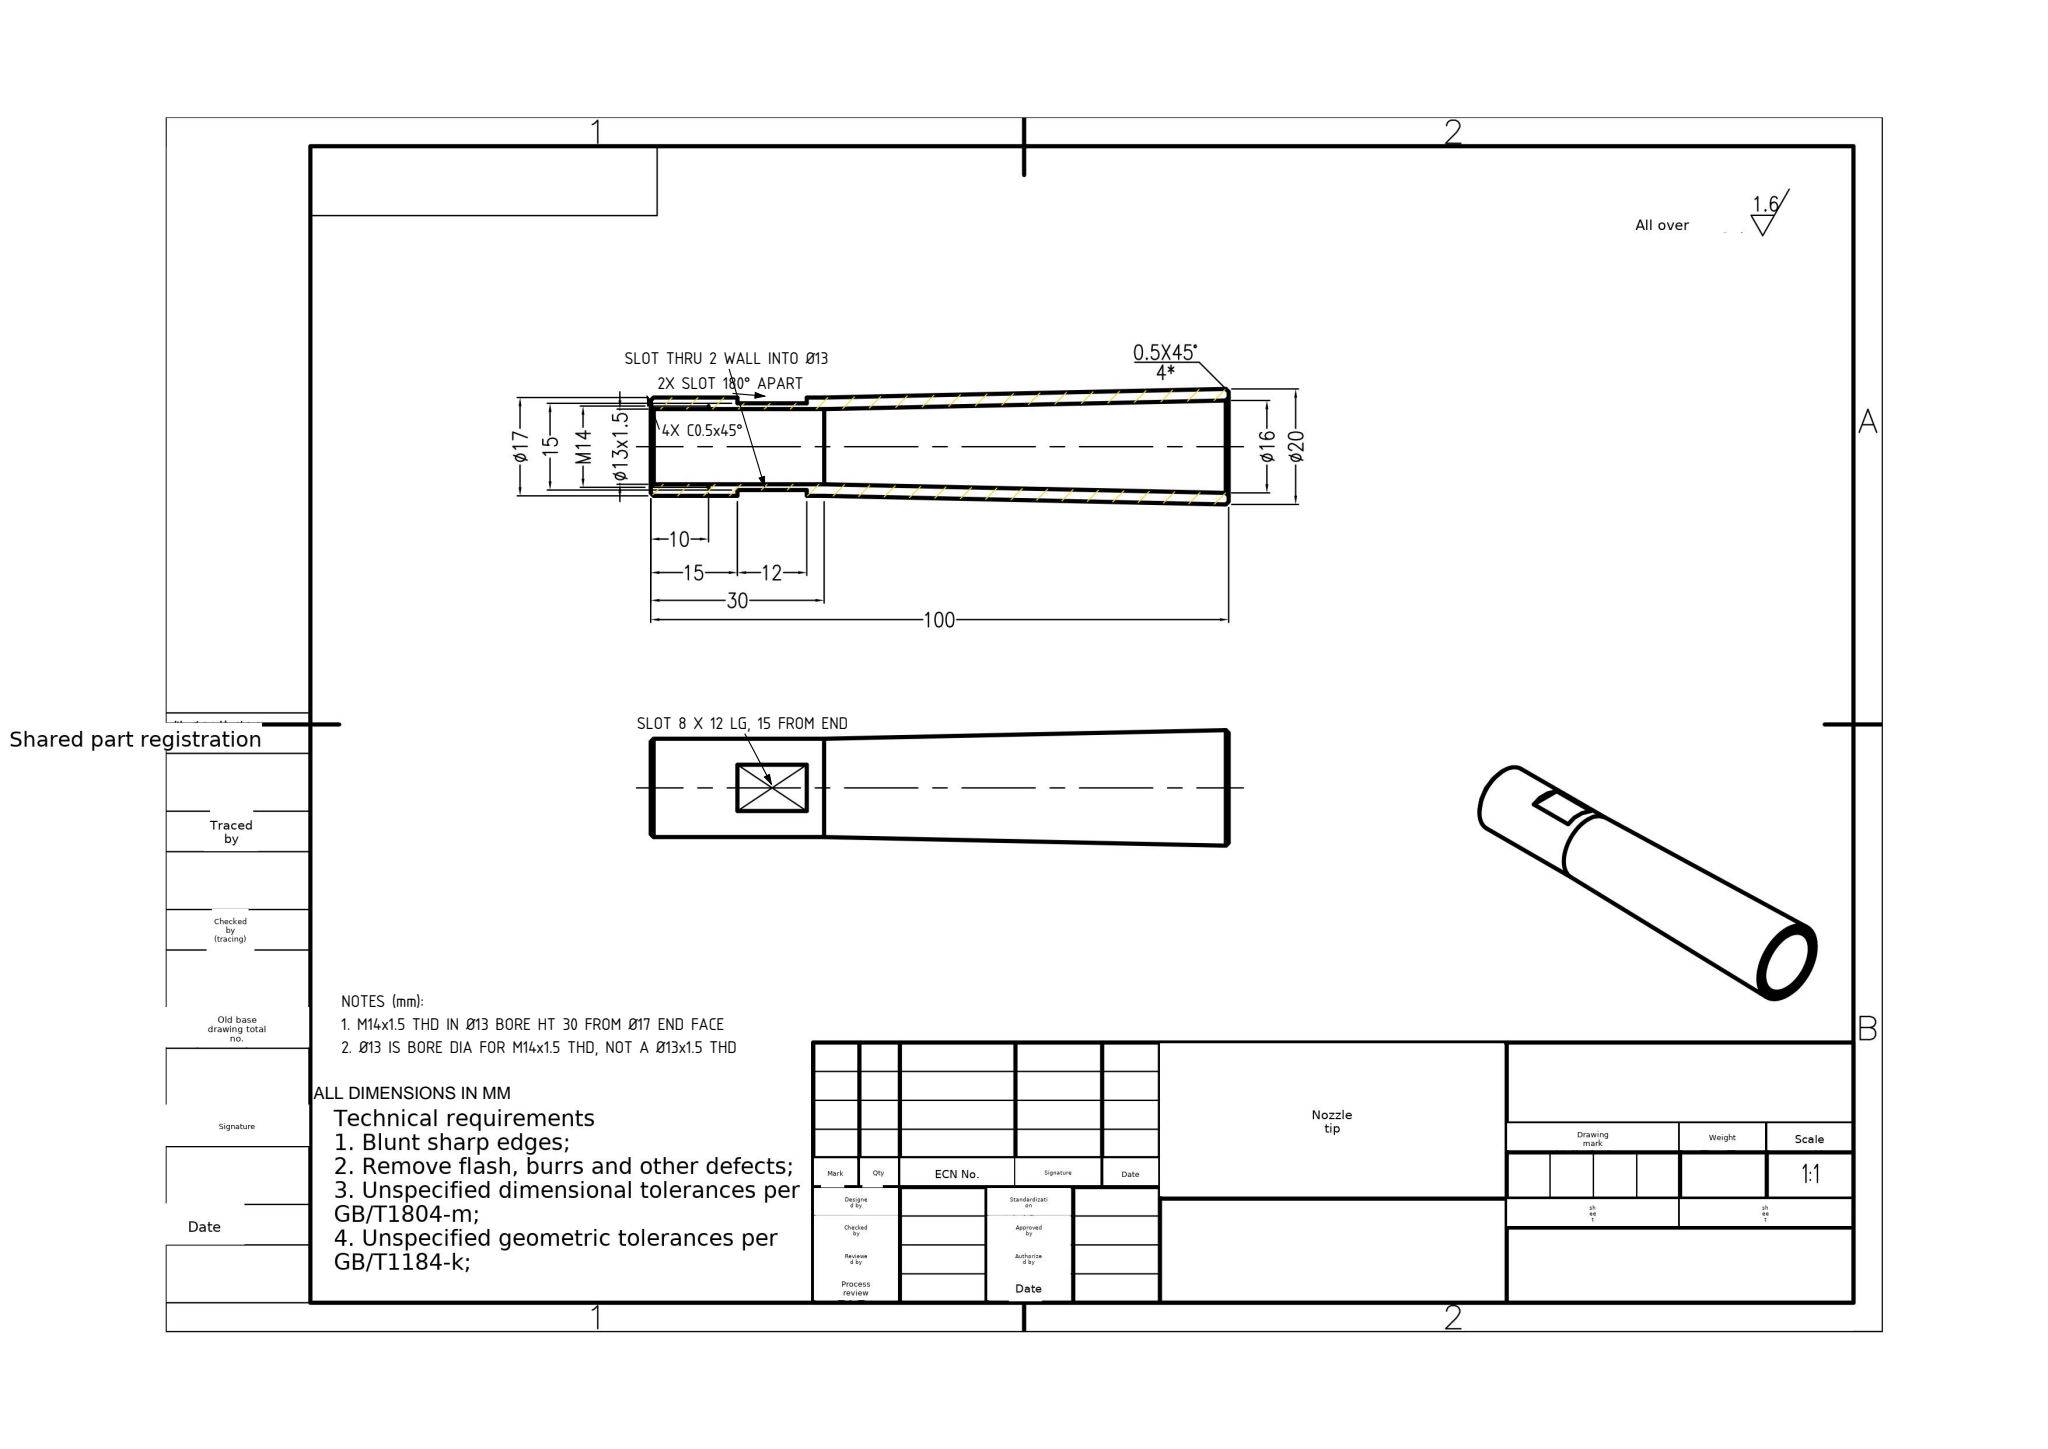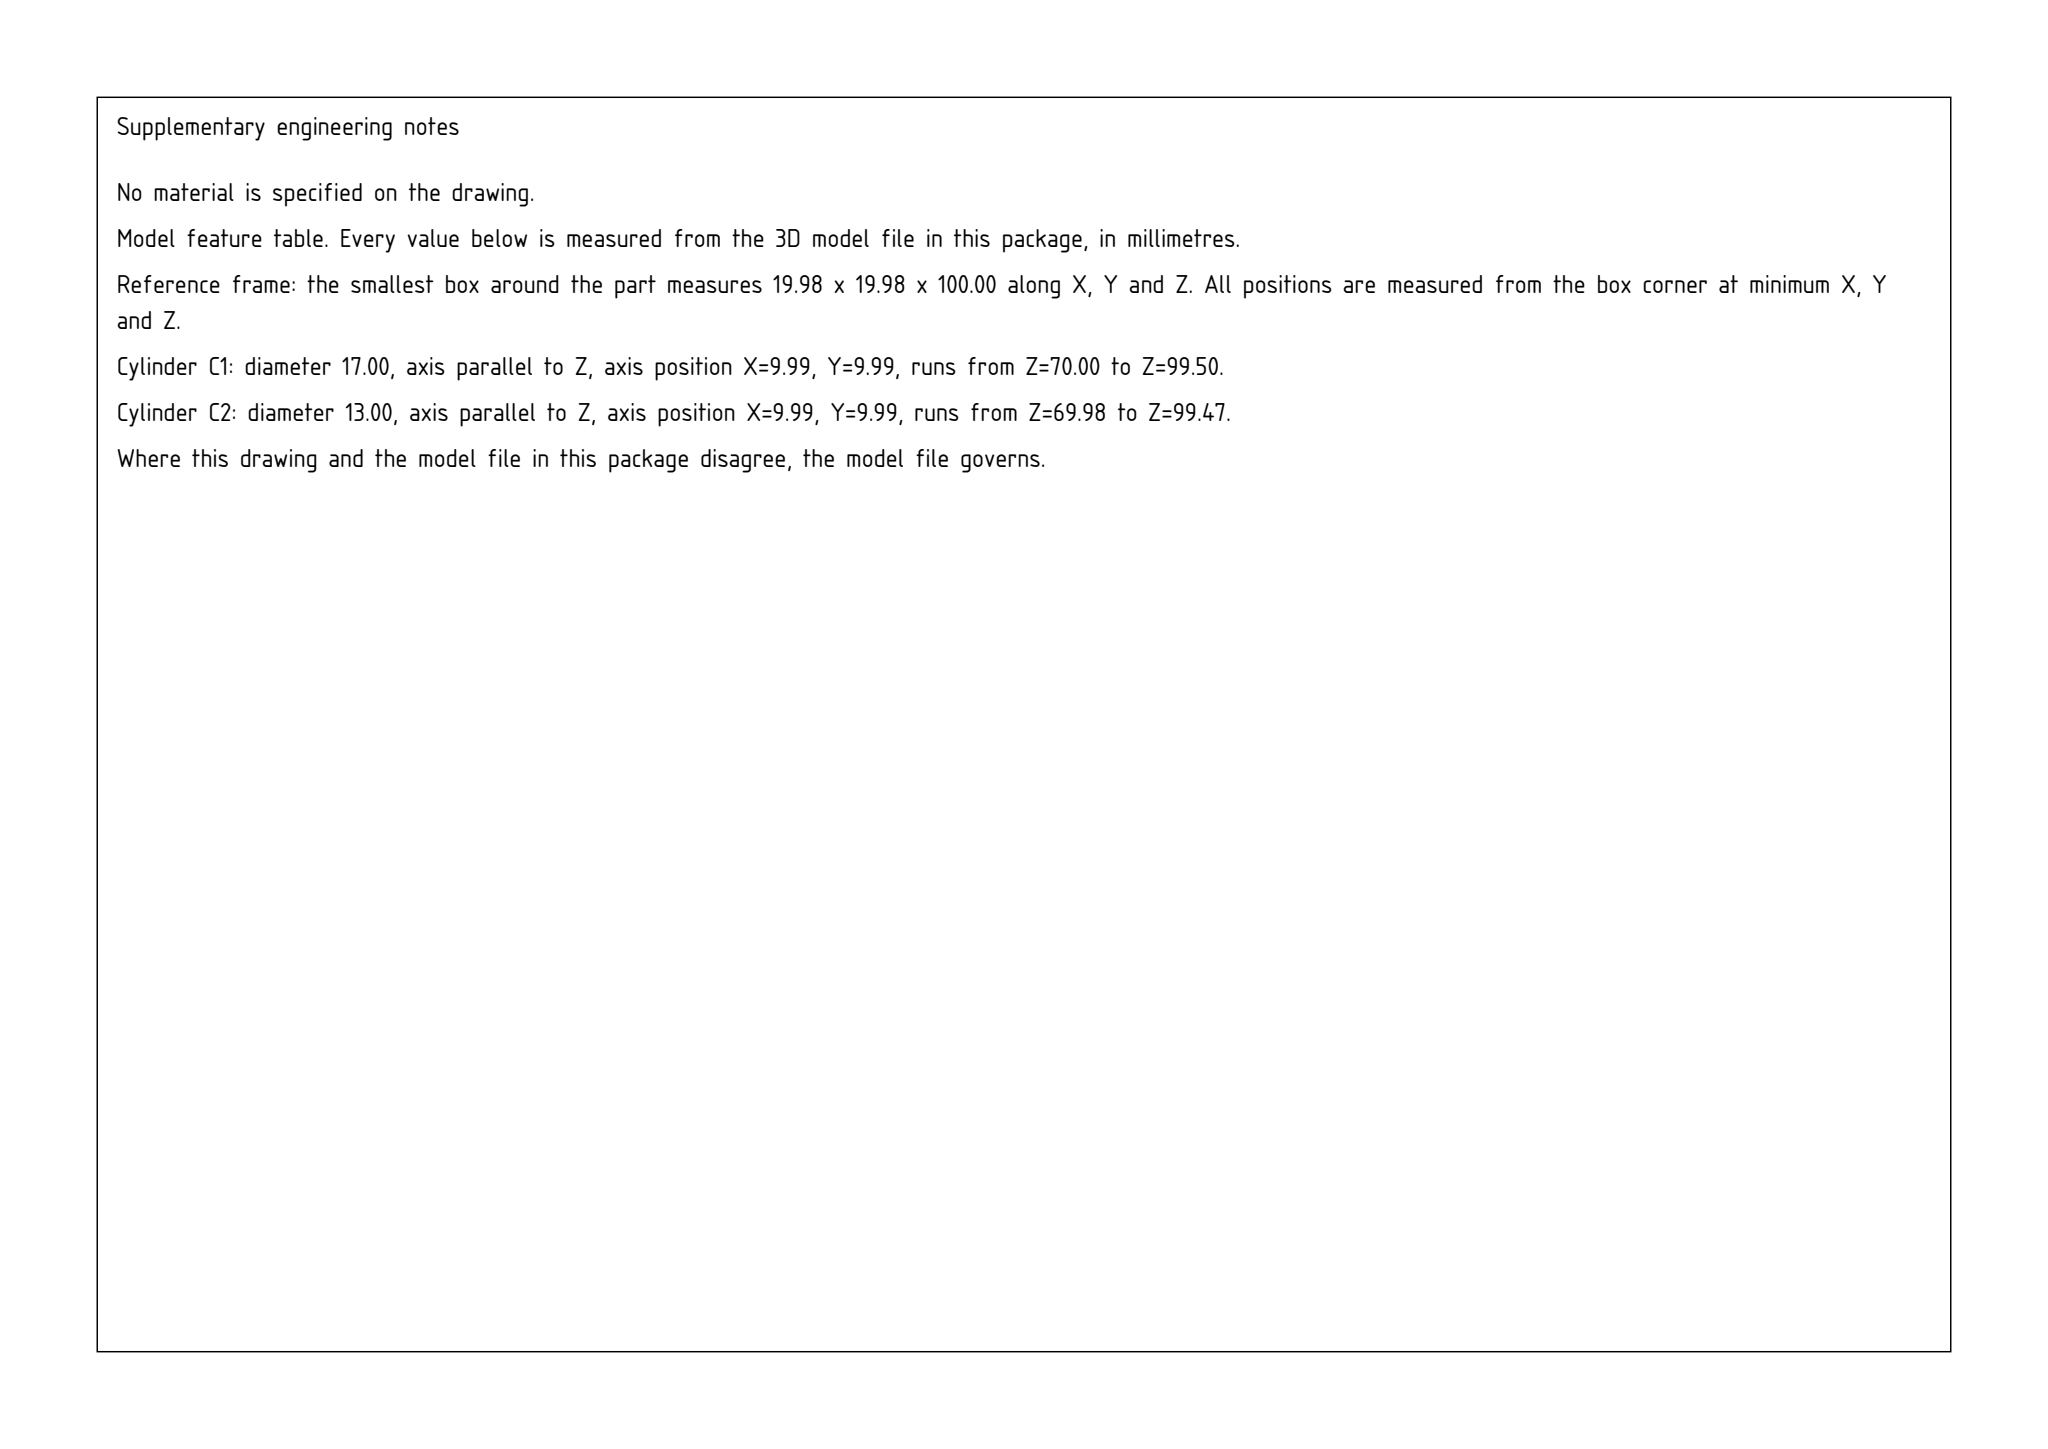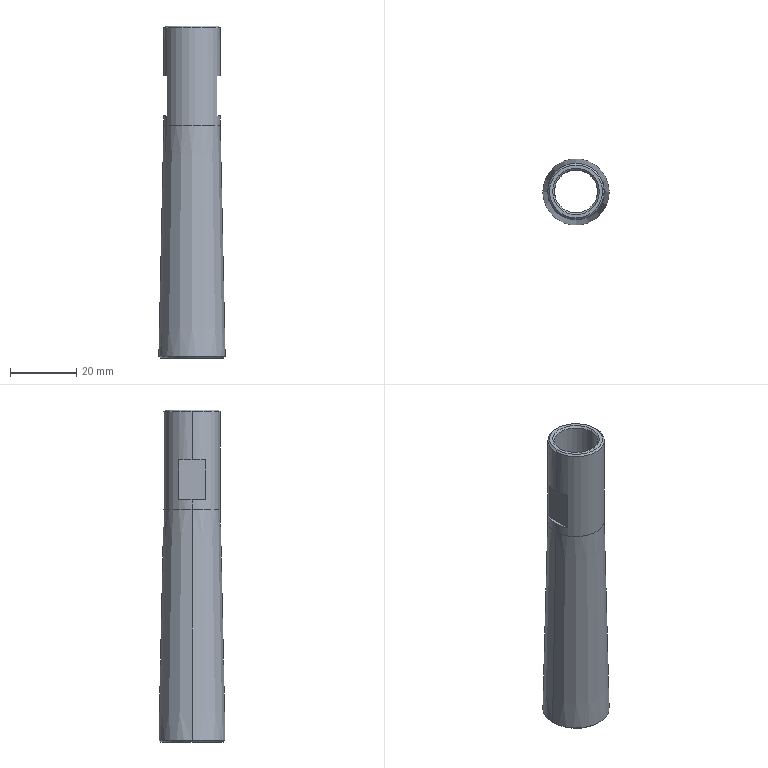Part | SolidWorks | mm | 1 solid | 24 faces | box 19.98 x 19.98 x 100 mm | volume 9930 mm3 | cone 12 | plane 8 | cylinder 4 | commonest cylinder face diameters 13 x2 17 x2
Drawing notes:
RECT SLOT 8 WIDE x 12 LG ON Ø17, 15 FROM Ø17 END FACE | from the solid: Planes x=2.5 & x=17.5, y 6-14 (8 wide), z 73-85 (12 lg); z=100 end face minus 85 = 15
SLOT: 2 PLCS, 180° APART ON Ø17 | from the solid: Two parallel slot walls at x=2.5 and x=17.5, both y 6-14, z 73-85, about axis x=y=10
SLOTS THRU 2 THK WALL INTO Ø13 BORE | from the solid: Ø17 OD and Ø13 bore (z 70-99.5) give 2 wall; slot end faces span x 1.5-2.5 and 17.5-18.5
M14x1.5 THD IN Ø13 BORE HT 30 FROM Ø17 END FACE | from the solid: hole/bore Ø13 z=70 to 99.5 with 0.5 chamfer to end face z=100; depth from face = 30
C0.5 x 45° 4 PLCS: OD & BORE, BOTH ENDS | from the solid: 90° cones ref Ø16 & Ø14.05 at z 99.5-100 and Ø19.98 & Ø17.02 at z 0-0.5, each 0.5 long
Ø13 IS BORE DIA FOR M14x1.5 THD, NOT A Ø13x1.5 THD | from the solid: Single cylindrical bore Ø13.0, z 70-99.5, no second thread feature in model
build123d program:
from build123d import *
from OCP.BRepFilletAPI import BRepFilletAPI_MakeChamfer

# Parameters (mm, degrees)
CUT_EXTRUDE2_DEPTH           = 20
CUT_EXTRUDE2_DEPTH_BACK      = 20
SKETCH4_W                    = 4.877
SKETCH4_H                    = 12
SKETCH4_W_2                  = 5.828
M14_TAPPED_HOLE1_D           = 12
M14_TAPPED_HOLE1_DEPTH       = 10
M14_TAPPED_HOLE1_CSINK_D     = 14.05
M14_TAPPED_HOLE1_CSINK_ANGLE = 90
M14_TAPPED_HOLE1_TIP         = 3.605
CHAMFER1_SIZE                = 0.5
CHAMFER1_SIZE2               = 0.5111
CHAMFER1_SIZE2_2             = 0.4896


with BuildPart() as part:
    # Sketch3 → Revolve1 (revolve)
    with BuildSketch(Plane(origin=(0, 0, 0), x_dir=(0, 0, -1), z_dir=(1, 0, 0)), mode=Mode.PRIVATE) as revolve1_sk:
        Polygon((0, 6.5), (0, 8.5), (30, 8.5), (100, 10), (100, 8), (30.021, 6.5), align=None)
    revolve(revolve1_sk.sketch.rotate(Axis((0, 0, 20.221), (0, 0, -1)), 90), axis=Axis((0, 0, 20.221), (0, 0, -1)))

    # Sketch4 → Cut-Extrude2 (cut, two sides: drawn at the far end of the back side and taken through both)
    with BuildSketch(Plane(origin=(0, 0, 0), x_dir=(1, 0, 0), z_dir=(0, 1, 0)).offset(-CUT_EXTRUDE2_DEPTH_BACK)):
        with Locations((-9.939, 21)):
            Rectangle(SKETCH4_W, SKETCH4_H)
        with Locations((10.414, 21)):
            Rectangle(SKETCH4_W_2, SKETCH4_H)
    extrude(amount=CUT_EXTRUDE2_DEPTH + CUT_EXTRUDE2_DEPTH_BACK, mode=Mode.SUBTRACT)

    # M14 Tapped Hole1
    with Locations(Plane.XY):
        with Locations((0, 0)):
            CounterSinkHole(M14_TAPPED_HOLE1_D / 2, M14_TAPPED_HOLE1_CSINK_D / 2, depth=M14_TAPPED_HOLE1_DEPTH, counter_sink_angle=M14_TAPPED_HOLE1_CSINK_ANGLE)
            with Locations((0, 0, -(M14_TAPPED_HOLE1_DEPTH + M14_TAPPED_HOLE1_TIP / 2))):  # 118° drill point
                Cone(0, M14_TAPPED_HOLE1_D / 2, M14_TAPPED_HOLE1_TIP, mode=Mode.SUBTRACT)

    # Chamfer1: one chamfer whose edges measure the first distance from different faces: ONE call of the kernel's chamfer builder (chamfer() names one face for all edges)
    chamfer1_edges_1 = [part.edges().sort_by_distance(p)[0] for p in [
        (-8.5, 0, 0),
    ]]
    chamfer1_edges_2 = [part.edges().sort_by_distance(p)[0] for p in [
        (-8, 0, -100),
    ]]
    chamfer1_side_2 = [part.faces().sort_by_distance(p)[0] for p in [
        (-7.25, 0, -65.011),
    ]]
    chamfer1_edges_3 = [part.edges().sort_by_distance(p)[0] for p in [
        (-10, 0, -100),
    ]]
    chamfer1_side_3 = [part.faces().sort_by_distance(p)[0] for p in [
        (-9.717, 0, -100),
    ]]
    chamfer1 = BRepFilletAPI_MakeChamfer(part.part.solid().wrapped)
    for e in chamfer1_edges_1:
        chamfer1.Add(CHAMFER1_SIZE, e.wrapped)
    for e in chamfer1_edges_2:
        chamfer1.Add(CHAMFER1_SIZE, CHAMFER1_SIZE2, e.wrapped, chamfer1_side_2[0].wrapped)  # the first distance lies on this face
    for e in chamfer1_edges_3:
        chamfer1.Add(CHAMFER1_SIZE, CHAMFER1_SIZE2_2, e.wrapped, chamfer1_side_3[0].wrapped)  # the first distance lies on this face
    add(Compound.cast(chamfer1.Shape()), mode=Mode.REPLACE)


solid = part.part
STEP:
#1=CARTESIAN_POINT('',(8.,0.,0.));
#2=VERTEX_POINT('',#1);
#3=CARTESIAN_POINT('',(-8.,0.,0.));
#4=VERTEX_POINT('',#3);
#5=CARTESIAN_POINT('',(0.,0.,0.));
#6=DIRECTION('',(0.,0.,1.));
#7=DIRECTION('',(-1.,0.,0.));
#8=AXIS2_PLACEMENT_3D('',#5,#6,#7);
#9=CIRCLE('',#8,8.);
#10=EDGE_CURVE('',#2,#4,#9,.T.);
#11=ORIENTED_EDGE('',*,*,#10,.F.);
#12=CARTESIAN_POINT('',(8.5,0.,-0.5));
#13=VERTEX_POINT('',#12);
#14=CARTESIAN_POINT('',(8.,0.,0.));
#15=DIRECTION('',(0.7071,0.,-0.7071));
#16=VECTOR('',#15,1000.);
#17=LINE('',#14,#16);
#18=EDGE_CURVE('',#2,#13,#17,.T.);
#19=ORIENTED_EDGE('',*,*,#18,.T.);
#20=CARTESIAN_POINT('',(-8.5,0.,-0.5));
#21=VERTEX_POINT('',#20);
#22=CARTESIAN_POINT('',(0.,0.,-0.5));
#23=DIRECTION('',(0.,0.,-1.));
#24=DIRECTION('',(-1.,0.,0.));
#25=AXIS2_PLACEMENT_3D('',#22,#23,#24);
#26=CIRCLE('',#25,8.5);
#27=EDGE_CURVE('',#21,#13,#26,.T.);
#28=ORIENTED_EDGE('',*,*,#27,.F.);
#29=CARTESIAN_POINT('',(-8.,0.,0.));
#30=DIRECTION('',(-0.7071,0.,-0.7071));
#31=VECTOR('',#30,1000.);
#32=LINE('',#29,#31);
#33=EDGE_CURVE('',#4,#21,#32,.T.);
#34=ORIENTED_EDGE('',*,*,#33,.F.);
#35=EDGE_LOOP('',(#11,#19,#28,#34));
#36=FACE_OUTER_BOUND('',#35,.T.);
#37=CARTESIAN_POINT('',(0.,0.,0.));
#38=DIRECTION('',(0.,0.,-1.));
#39=DIRECTION('',(-1.,0.,0.));
#40=AXIS2_PLACEMENT_3D('',#37,#38,#39);
#41=CONICAL_SURFACE('',#40,8.,0.7854);
#42=ADVANCED_FACE('',(#36),#41,.T.);
#43=CARTESIAN_POINT('',(-9.5,0.,-100.));
#44=VERTEX_POINT('',#43);
#45=CARTESIAN_POINT('',(9.5,0.,-100.));
#46=VERTEX_POINT('',#45);
#47=CARTESIAN_POINT('',(0.,0.,-100.));
#48=DIRECTION('',(0.,0.,-1.));
#49=DIRECTION('',(1.,0.,0.));
#50=AXIS2_PLACEMENT_3D('',#47,#48,#49);
#51=CIRCLE('',#50,9.5);
#52=EDGE_CURVE('',#44,#46,#51,.T.);
#53=ORIENTED_EDGE('',*,*,#52,.F.);
#54=CARTESIAN_POINT('',(-9.99,0.,-99.51));
#55=VERTEX_POINT('',#54);
#56=CARTESIAN_POINT('',(-9.99,0.,-99.51));
#57=DIRECTION('',(-0.7071,0.,0.7071));
#58=VECTOR('',#57,1000.);
#59=LINE('',#56,#58);
#60=EDGE_CURVE('',#44,#55,#59,.T.);
#61=ORIENTED_EDGE('',*,*,#60,.T.);
#62=CARTESIAN_POINT('',(9.99,0.,-99.51));
#63=VERTEX_POINT('',#62);
#64=CARTESIAN_POINT('',(0.,0.,-99.51));
#65=DIRECTION('',(0.,0.,1.));
#66=DIRECTION('',(1.,0.,0.));
#67=AXIS2_PLACEMENT_3D('',#64,#65,#66);
#68=CIRCLE('',#67,9.99);
#69=EDGE_CURVE('',#63,#55,#68,.T.);
#70=ORIENTED_EDGE('',*,*,#69,.F.);
#71=CARTESIAN_POINT('',(9.99,0.,-99.51));
#72=DIRECTION('',(0.7071,0.,0.7071));
#73=VECTOR('',#72,1000.);
#74=LINE('',#71,#73);
#75=EDGE_CURVE('',#46,#63,#74,.T.);
#76=ORIENTED_EDGE('',*,*,#75,.F.);
#77=EDGE_LOOP('',(#53,#61,#70,#76));
#78=FACE_OUTER_BOUND('',#77,.T.);
#79=CARTESIAN_POINT('',(0.,0.,-99.51));
#80=DIRECTION('',(0.,0.,1.));
#81=DIRECTION('',(1.,0.,0.));
#82=AXIS2_PLACEMENT_3D('',#79,#80,#81);
#83=CONICAL_SURFACE('',#82,9.99,0.7854);
#84=ADVANCED_FACE('',(#78),#83,.T.);
#85=CARTESIAN_POINT('',(7.989,0.,-99.5));
#86=VERTEX_POINT('',#85);
#87=CARTESIAN_POINT('',(-7.989,0.,-99.5));
#88=VERTEX_POINT('',#87);
#89=CARTESIAN_POINT('',(0.,0.,-99.5));
#90=DIRECTION('',(0.,0.,-1.));
#91=DIRECTION('',(1.,0.,0.));
#92=AXIS2_PLACEMENT_3D('',#89,#90,#91);
#93=CIRCLE('',#92,7.989);
#94=EDGE_CURVE('',#86,#88,#93,.T.);
#95=ORIENTED_EDGE('',*,*,#94,.F.);
#96=CARTESIAN_POINT('',(8.511,0.,-100.));
#97=VERTEX_POINT('',#96);
#98=CARTESIAN_POINT('',(8.511,0.,-100.));
#99=DIRECTION('',(0.7221,0.,-0.6918));
#100=VECTOR('',#99,1000.);
#101=LINE('',#98,#100);
#102=EDGE_CURVE('',#86,#97,#101,.T.);
#103=ORIENTED_EDGE('',*,*,#102,.T.);
#104=CARTESIAN_POINT('',(-8.511,0.,-100.));
#105=VERTEX_POINT('',#104);
#106=CARTESIAN_POINT('',(0.,0.,-100.));
#107=DIRECTION('',(0.,0.,1.));
#108=DIRECTION('',(1.,0.,0.));
#109=AXIS2_PLACEMENT_3D('',#106,#107,#108);
#110=CIRCLE('',#109,8.511);
#111=EDGE_CURVE('',#105,#97,#110,.T.);
#112=ORIENTED_EDGE('',*,*,#111,.F.);
#113=CARTESIAN_POINT('',(-8.511,0.,-100.));
#114=DIRECTION('',(-0.7221,0.,-0.6918));
#115=VECTOR('',#114,1000.);
#116=LINE('',#113,#115);
#117=EDGE_CURVE('',#88,#105,#116,.T.);
#118=ORIENTED_EDGE('',*,*,#117,.F.);
#119=EDGE_LOOP('',(#95,#103,#112,#118));
#120=FACE_OUTER_BOUND('',#119,.T.);
#121=CARTESIAN_POINT('',(0.,0.,-100.));
#122=DIRECTION('',(0.,0.,-1.));
#123=DIRECTION('',(-1.,0.,0.));
#124=AXIS2_PLACEMENT_3D('',#121,#122,#123);
#125=CONICAL_SURFACE('',#124,8.511,0.8068);
#126=ADVANCED_FACE('',(#120),#125,.F.);
#127=CARTESIAN_POINT('',(-6.5,0.,-0.525));
#128=VERTEX_POINT('',#127);
#129=CARTESIAN_POINT('',(6.5,0.,-0.525));
#130=VERTEX_POINT('',#129);
#131=CARTESIAN_POINT('',(0.,0.,-0.525));
#132=DIRECTION('',(0.,0.,1.));
#133=DIRECTION('',(1.,0.,0.));
#134=AXIS2_PLACEMENT_3D('',#131,#132,#133);
#135=CIRCLE('',#134,6.5);
#136=EDGE_CURVE('',#128,#130,#135,.T.);
#137=ORIENTED_EDGE('',*,*,#136,.F.);
#138=CARTESIAN_POINT('',(-7.025,0.,-0.));
#139=VERTEX_POINT('',#138);
#140=CARTESIAN_POINT('',(-7.025,0.,-0.));
#141=DIRECTION('',(-0.7071,0.,0.7071));
#142=VECTOR('',#141,1000.);
#143=LINE('',#140,#142);
#144=EDGE_CURVE('',#128,#139,#143,.T.);
#145=ORIENTED_EDGE('',*,*,#144,.T.);
#146=CARTESIAN_POINT('',(7.025,0.,-0.));
#147=VERTEX_POINT('',#146);
#148=CARTESIAN_POINT('',(0.,0.,-0.));
#149=DIRECTION('',(0.,0.,1.));
#150=DIRECTION('',(1.,0.,0.));
#151=AXIS2_PLACEMENT_3D('',#148,#149,#150);
#152=CIRCLE('',#151,7.025);
#153=EDGE_CURVE('',#139,#147,#152,.T.);
#154=ORIENTED_EDGE('',*,*,#153,.T.);
#155=CARTESIAN_POINT('',(7.025,0.,-0.));
#156=DIRECTION('',(0.7071,0.,0.7071));
#157=VECTOR('',#156,1000.);
#158=LINE('',#155,#157);
#159=EDGE_CURVE('',#130,#147,#158,.T.);
#160=ORIENTED_EDGE('',*,*,#159,.F.);
#161=EDGE_LOOP('',(#137,#145,#154,#160));
#162=FACE_OUTER_BOUND('',#161,.T.);
#163=CARTESIAN_POINT('',(0.,0.,-0.));
#164=DIRECTION('',(0.,0.,1.));
#165=DIRECTION('',(1.,0.,0.));
#166=AXIS2_PLACEMENT_3D('',#163,#164,#165);
#167=CONICAL_SURFACE('',#166,7.025,0.7854);
#168=ADVANCED_FACE('',(#162),#167,.F.);
#169=CARTESIAN_POINT('',(-6.5,0.,-30.021));
#170=VERTEX_POINT('',#169);
#171=CARTESIAN_POINT('',(6.5,0.,-30.021));
#172=VERTEX_POINT('',#171);
#173=CARTESIAN_POINT('',(0.,0.,-30.021));
#174=DIRECTION('',(0.,0.,1.));
#175=DIRECTION('',(1.,0.,0.));
#176=AXIS2_PLACEMENT_3D('',#173,#174,#175);
#177=CIRCLE('',#176,6.5);
#178=EDGE_CURVE('',#170,#172,#177,.T.);
#179=ORIENTED_EDGE('',*,*,#178,.F.);
#180=CARTESIAN_POINT('',(-6.5,0.,20.221));
#181=DIRECTION('',(0.,0.,1.));
#182=VECTOR('',#181,1000.);
#183=LINE('',#180,#182);
#184=EDGE_CURVE('',#170,#128,#183,.T.);
#185=ORIENTED_EDGE('',*,*,#184,.T.);
#186=ORIENTED_EDGE('',*,*,#136,.T.);
#187=CARTESIAN_POINT('',(6.5,0.,20.221));
#188=DIRECTION('',(0.,0.,1.));
#189=VECTOR('',#188,1000.);
#190=LINE('',#187,#189);
#191=EDGE_CURVE('',#172,#130,#190,.T.);
#192=ORIENTED_EDGE('',*,*,#191,.F.);
#193=EDGE_LOOP('',(#179,#185,#186,#192));
#194=FACE_OUTER_BOUND('',#193,.T.);
#195=CARTESIAN_POINT('',(0.,0.,20.221));
#196=DIRECTION('',(0.,0.,1.));
#197=DIRECTION('',(1.,0.,0.));
#198=AXIS2_PLACEMENT_3D('',#195,#196,#197);
#199=CYLINDRICAL_SURFACE('',#198,6.5);
#200=ADVANCED_FACE('',(#194),#199,.F.);
#201=ORIENTED_EDGE('',*,*,#178,.T.);
#202=CARTESIAN_POINT('',(6.5,0.,-30.021));
#203=DIRECTION('',(0.02142,0.,-0.9998));
#204=VECTOR('',#203,1000.);
#205=LINE('',#202,#204);
#206=EDGE_CURVE('',#172,#86,#205,.T.);
#207=ORIENTED_EDGE('',*,*,#206,.T.);
#208=ORIENTED_EDGE('',*,*,#94,.T.);
#209=CARTESIAN_POINT('',(-6.5,0.,-30.021));
#210=DIRECTION('',(-0.02142,0.,-0.9998));
#211=VECTOR('',#210,1000.);
#212=LINE('',#209,#211);
#213=EDGE_CURVE('',#170,#88,#212,.T.);
#214=ORIENTED_EDGE('',*,*,#213,.F.);
#215=EDGE_LOOP('',(#201,#207,#208,#214));
#216=FACE_OUTER_BOUND('',#215,.T.);
#217=CARTESIAN_POINT('',(0.,0.,-30.021));
#218=DIRECTION('',(0.,0.,-1.));
#219=DIRECTION('',(-1.,0.,0.));
#220=AXIS2_PLACEMENT_3D('',#217,#218,#219);
#221=CONICAL_SURFACE('',#220,6.5,0.02143);
#222=ADVANCED_FACE('',(#216),#221,.F.);
#223=CARTESIAN_POINT('',(8.5,0.,-30.));
#224=VERTEX_POINT('',#223);
#225=CARTESIAN_POINT('',(-8.5,0.,-30.));
#226=VERTEX_POINT('',#225);
#227=CARTESIAN_POINT('',(0.,0.,-30.));
#228=DIRECTION('',(0.,0.,1.));
#229=DIRECTION('',(1.,0.,0.));
#230=AXIS2_PLACEMENT_3D('',#227,#228,#229);
#231=CIRCLE('',#230,8.5);
#232=EDGE_CURVE('',#224,#226,#231,.T.);
#233=ORIENTED_EDGE('',*,*,#232,.F.);
#234=CARTESIAN_POINT('',(10.,0.,-100.));
#235=DIRECTION('',(0.02142,0.,-0.9998));
#236=VECTOR('',#235,1000.);
#237=LINE('',#234,#236);
#238=EDGE_CURVE('',#224,#63,#237,.T.);
#239=ORIENTED_EDGE('',*,*,#238,.T.);
#240=ORIENTED_EDGE('',*,*,#69,.T.);
#241=CARTESIAN_POINT('',(-10.,0.,-100.));
#242=DIRECTION('',(-0.02142,0.,-0.9998));
#243=VECTOR('',#242,1000.);
#244=LINE('',#241,#243);
#245=EDGE_CURVE('',#226,#55,#244,.T.);
#246=ORIENTED_EDGE('',*,*,#245,.F.);
#247=EDGE_LOOP('',(#233,#239,#240,#246));
#248=FACE_OUTER_BOUND('',#247,.T.);
#249=CARTESIAN_POINT('',(0.,0.,-100.));
#250=DIRECTION('',(0.,0.,-1.));
#251=DIRECTION('',(-1.,0.,0.));
#252=AXIS2_PLACEMENT_3D('',#249,#250,#251);
#253=CONICAL_SURFACE('',#252,10.,0.02143);
#254=ADVANCED_FACE('',(#248),#253,.T.);
#255=ORIENTED_EDGE('',*,*,#232,.T.);
#256=CARTESIAN_POINT('',(-8.5,0.,-27.));
#257=VERTEX_POINT('',#256);
#258=CARTESIAN_POINT('',(-8.5,0.,20.221));
#259=DIRECTION('',(0.,0.,1.));
#260=VECTOR('',#259,1000.);
#261=LINE('',#258,#260);
#262=EDGE_CURVE('',#226,#257,#261,.T.);
#263=ORIENTED_EDGE('',*,*,#262,.T.);
#264=CARTESIAN_POINT('',(-7.5,4.,-27.));
#265=VERTEX_POINT('',#264);
#266=CARTESIAN_POINT('',(0.,0.,-27.));
#267=DIRECTION('',(0.,0.,1.));
#268=DIRECTION('',(1.,0.,-0.));
#269=AXIS2_PLACEMENT_3D('',#266,#267,#268);
#270=CIRCLE('',#269,8.5);
#271=EDGE_CURVE('',#265,#257,#270,.T.);
#272=ORIENTED_EDGE('',*,*,#271,.F.);
#273=CARTESIAN_POINT('',(-7.5,4.,-15.));
#274=VERTEX_POINT('',#273);
#275=CARTESIAN_POINT('',(-7.5,4.,20.221));
#276=DIRECTION('',(0.,0.,-1.));
#277=VECTOR('',#276,1000.);
#278=LINE('',#275,#277);
#279=EDGE_CURVE('',#274,#265,#278,.T.);
#280=ORIENTED_EDGE('',*,*,#279,.F.);
#281=CARTESIAN_POINT('',(-8.5,0.,-15.));
#282=VERTEX_POINT('',#281);
#283=CARTESIAN_POINT('',(0.,0.,-15.));
#284=DIRECTION('',(0.,0.,-1.));
#285=DIRECTION('',(-1.,0.,0.));
#286=AXIS2_PLACEMENT_3D('',#283,#284,#285);
#287=CIRCLE('',#286,8.5);
#288=EDGE_CURVE('',#282,#274,#287,.T.);
#289=ORIENTED_EDGE('',*,*,#288,.F.);
#290=CARTESIAN_POINT('',(-8.5,0.,20.221));
#291=DIRECTION('',(0.,0.,1.));
#292=VECTOR('',#291,1000.);
#293=LINE('',#290,#292);
#294=EDGE_CURVE('',#282,#21,#293,.T.);
#295=ORIENTED_EDGE('',*,*,#294,.T.);
#296=ORIENTED_EDGE('',*,*,#27,.T.);
#297=CARTESIAN_POINT('',(8.5,0.,-15.));
#298=VERTEX_POINT('',#297);
#299=CARTESIAN_POINT('',(8.5,0.,20.221));
#300=DIRECTION('',(0.,0.,1.));
#301=VECTOR('',#300,1000.);
#302=LINE('',#299,#301);
#303=EDGE_CURVE('',#298,#13,#302,.T.);
#304=ORIENTED_EDGE('',*,*,#303,.F.);
#305=CARTESIAN_POINT('',(7.5,4.,-15.));
#306=VERTEX_POINT('',#305);
#307=CARTESIAN_POINT('',(0.,0.,-15.));
#308=DIRECTION('',(0.,0.,-1.));
#309=DIRECTION('',(-1.,0.,0.));
#310=AXIS2_PLACEMENT_3D('',#307,#308,#309);
#311=CIRCLE('',#310,8.5);
#312=EDGE_CURVE('',#306,#298,#311,.T.);
#313=ORIENTED_EDGE('',*,*,#312,.F.);
#314=CARTESIAN_POINT('',(7.5,4.,-27.));
#315=VERTEX_POINT('',#314);
#316=CARTESIAN_POINT('',(7.5,4.,20.221));
#317=DIRECTION('',(0.,0.,1.));
#318=VECTOR('',#317,1000.);
#319=LINE('',#316,#318);
#320=EDGE_CURVE('',#315,#306,#319,.T.);
#321=ORIENTED_EDGE('',*,*,#320,.F.);
#322=CARTESIAN_POINT('',(8.5,0.,-27.));
#323=VERTEX_POINT('',#322);
#324=CARTESIAN_POINT('',(0.,0.,-27.));
#325=DIRECTION('',(0.,0.,1.));
#326=DIRECTION('',(1.,0.,0.));
#327=AXIS2_PLACEMENT_3D('',#324,#325,#326);
#328=CIRCLE('',#327,8.5);
#329=EDGE_CURVE('',#323,#315,#328,.T.);
#330=ORIENTED_EDGE('',*,*,#329,.F.);
#331=CARTESIAN_POINT('',(8.5,0.,20.221));
#332=DIRECTION('',(0.,0.,1.));
#333=VECTOR('',#332,1000.);
#334=LINE('',#331,#333);
#335=EDGE_CURVE('',#224,#323,#334,.T.);
#336=ORIENTED_EDGE('',*,*,#335,.F.);
#337=EDGE_LOOP('',(#255,#263,#272,#280,#289,#295,#296,#304,#313,#321,#330,#336));
#338=FACE_OUTER_BOUND('',#337,.T.);
#339=CARTESIAN_POINT('',(0.,0.,20.221));
#340=DIRECTION('',(0.,0.,1.));
#341=DIRECTION('',(1.,0.,0.));
#342=AXIS2_PLACEMENT_3D('',#339,#340,#341);
#343=CYLINDRICAL_SURFACE('',#342,8.5);
#344=ADVANCED_FACE('',(#338),#343,.T.);
#345=ORIENTED_EDGE('',*,*,#262,.F.);
#346=CARTESIAN_POINT('',(0.,0.,-30.));
#347=DIRECTION('',(0.,0.,1.));
#348=DIRECTION('',(1.,0.,0.));
#349=AXIS2_PLACEMENT_3D('',#346,#347,#348);
#350=CIRCLE('',#349,8.5);
#351=EDGE_CURVE('',#226,#224,#350,.T.);
#352=ORIENTED_EDGE('',*,*,#351,.T.);
#353=ORIENTED_EDGE('',*,*,#335,.T.);
#354=CARTESIAN_POINT('',(7.5,-4.,-27.));
#355=VERTEX_POINT('',#354);
#356=CARTESIAN_POINT('',(0.,0.,-27.));
#357=DIRECTION('',(0.,0.,1.));
#358=DIRECTION('',(1.,0.,0.));
#359=AXIS2_PLACEMENT_3D('',#356,#357,#358);
#360=CIRCLE('',#359,8.5);
#361=EDGE_CURVE('',#355,#323,#360,.T.);
#362=ORIENTED_EDGE('',*,*,#361,.F.);
#363=CARTESIAN_POINT('',(7.5,-4.,-15.));
#364=VERTEX_POINT('',#363);
#365=CARTESIAN_POINT('',(7.5,-4.,20.221));
#366=DIRECTION('',(0.,0.,-1.));
#367=VECTOR('',#366,1000.);
#368=LINE('',#365,#367);
#369=EDGE_CURVE('',#364,#355,#368,.T.);
#370=ORIENTED_EDGE('',*,*,#369,.F.);
#371=CARTESIAN_POINT('',(0.,0.,-15.));
#372=DIRECTION('',(0.,0.,-1.));
#373=DIRECTION('',(-1.,0.,0.));
#374=AXIS2_PLACEMENT_3D('',#371,#372,#373);
#375=CIRCLE('',#374,8.5);
#376=EDGE_CURVE('',#298,#364,#375,.T.);
#377=ORIENTED_EDGE('',*,*,#376,.F.);
#378=ORIENTED_EDGE('',*,*,#303,.T.);
#379=CARTESIAN_POINT('',(0.,0.,-0.5));
#380=DIRECTION('',(0.,0.,-1.));
#381=DIRECTION('',(-1.,0.,0.));
#382=AXIS2_PLACEMENT_3D('',#379,#380,#381);
#383=CIRCLE('',#382,8.5);
#384=EDGE_CURVE('',#13,#21,#383,.T.);
#385=ORIENTED_EDGE('',*,*,#384,.T.);
#386=ORIENTED_EDGE('',*,*,#294,.F.);
#387=CARTESIAN_POINT('',(-7.5,-4.,-15.));
#388=VERTEX_POINT('',#387);
#389=CARTESIAN_POINT('',(0.,0.,-15.));
#390=DIRECTION('',(0.,0.,-1.));
#391=DIRECTION('',(-1.,0.,0.));
#392=AXIS2_PLACEMENT_3D('',#389,#390,#391);
#393=CIRCLE('',#392,8.5);
#394=EDGE_CURVE('',#388,#282,#393,.T.);
#395=ORIENTED_EDGE('',*,*,#394,.F.);
#396=CARTESIAN_POINT('',(-7.5,-4.,-27.));
#397=VERTEX_POINT('',#396);
#398=CARTESIAN_POINT('',(-7.5,-4.,20.221));
#399=DIRECTION('',(0.,0.,1.));
#400=VECTOR('',#399,1000.);
#401=LINE('',#398,#400);
#402=EDGE_CURVE('',#397,#388,#401,.T.);
#403=ORIENTED_EDGE('',*,*,#402,.F.);
#404=CARTESIAN_POINT('',(0.,0.,-27.));
#405=DIRECTION('',(0.,0.,1.));
#406=DIRECTION('',(1.,0.,-0.));
#407=AXIS2_PLACEMENT_3D('',#404,#405,#406);
#408=CIRCLE('',#407,8.5);
#409=EDGE_CURVE('',#257,#397,#408,.T.);
#410=ORIENTED_EDGE('',*,*,#409,.F.);
#411=EDGE_LOOP('',(#345,#352,#353,#362,#370,#377,#378,#385,#386,#395,#403,#410));
#412=FACE_OUTER_BOUND('',#411,.T.);
#413=CARTESIAN_POINT('',(0.,0.,20.221));
#414=DIRECTION('',(0.,0.,1.));
#415=DIRECTION('',(1.,0.,0.));
#416=AXIS2_PLACEMENT_3D('',#413,#414,#415);
#417=CYLINDRICAL_SURFACE('',#416,8.5);
#418=ADVANCED_FACE('',(#412),#417,.T.);
#419=ORIENTED_EDGE('',*,*,#238,.F.);
#420=ORIENTED_EDGE('',*,*,#351,.F.);
#421=ORIENTED_EDGE('',*,*,#245,.T.);
#422=CARTESIAN_POINT('',(0.,0.,-99.51));
#423=DIRECTION('',(0.,0.,1.));
#424=DIRECTION('',(1.,0.,0.));
#425=AXIS2_PLACEMENT_3D('',#422,#423,#424);
#426=CIRCLE('',#425,9.99);
#427=EDGE_CURVE('',#55,#63,#426,.T.);
#428=ORIENTED_EDGE('',*,*,#427,.T.);
#429=EDGE_LOOP('',(#419,#420,#421,#428));
#430=FACE_OUTER_BOUND('',#429,.T.);
#431=CARTESIAN_POINT('',(0.,0.,-100.));
#432=DIRECTION('',(0.,0.,-1.));
#433=DIRECTION('',(-1.,0.,0.));
#434=AXIS2_PLACEMENT_3D('',#431,#432,#433);
#435=CONICAL_SURFACE('',#434,10.,0.02143);
#436=ADVANCED_FACE('',(#430),#435,.T.);
#437=ORIENTED_EDGE('',*,*,#111,.T.);
#438=CARTESIAN_POINT('',(0.,0.,-100.));
#439=DIRECTION('',(0.,0.,1.));
#440=DIRECTION('',(1.,0.,0.));
#441=AXIS2_PLACEMENT_3D('',#438,#439,#440);
#442=CIRCLE('',#441,8.511);
#443=EDGE_CURVE('',#97,#105,#442,.T.);
#444=ORIENTED_EDGE('',*,*,#443,.T.);
#445=EDGE_LOOP('',(#437,#444));
#446=FACE_BOUND('',#445,.T.);
#447=CARTESIAN_POINT('',(0.,0.,-100.));
#448=DIRECTION('',(0.,0.,-1.));
#449=DIRECTION('',(1.,0.,0.));
#450=AXIS2_PLACEMENT_3D('',#447,#448,#449);
#451=CIRCLE('',#450,9.5);
#452=EDGE_CURVE('',#46,#44,#451,.T.);
#453=ORIENTED_EDGE('',*,*,#452,.T.);
#454=ORIENTED_EDGE('',*,*,#52,.T.);
#455=EDGE_LOOP('',(#453,#454));
#456=FACE_OUTER_BOUND('',#455,.T.);
#457=CARTESIAN_POINT('',(0.,10.,-100.));
#458=DIRECTION('',(0.,0.,1.));
#459=DIRECTION('',(1.,0.,0.));
#460=AXIS2_PLACEMENT_3D('',#457,#458,#459);
#461=PLANE('',#460);
#462=ADVANCED_FACE('',(#446,#456),#461,.F.);
#463=ORIENTED_EDGE('',*,*,#206,.F.);
#464=CARTESIAN_POINT('',(0.,0.,-30.021));
#465=DIRECTION('',(0.,0.,1.));
#466=DIRECTION('',(1.,0.,0.));
#467=AXIS2_PLACEMENT_3D('',#464,#465,#466);
#468=CIRCLE('',#467,6.5);
#469=EDGE_CURVE('',#172,#170,#468,.T.);
#470=ORIENTED_EDGE('',*,*,#469,.T.);
#471=ORIENTED_EDGE('',*,*,#213,.T.);
#472=CARTESIAN_POINT('',(0.,0.,-99.5));
#473=DIRECTION('',(0.,0.,-1.));
#474=DIRECTION('',(1.,0.,0.));
#475=AXIS2_PLACEMENT_3D('',#472,#473,#474);
#476=CIRCLE('',#475,7.989);
#477=EDGE_CURVE('',#88,#86,#476,.T.);
#478=ORIENTED_EDGE('',*,*,#477,.T.);
#479=EDGE_LOOP('',(#463,#470,#471,#478));
#480=FACE_OUTER_BOUND('',#479,.T.);
#481=CARTESIAN_POINT('',(0.,0.,-30.021));
#482=DIRECTION('',(0.,0.,-1.));
#483=DIRECTION('',(-1.,0.,0.));
#484=AXIS2_PLACEMENT_3D('',#481,#482,#483);
#485=CONICAL_SURFACE('',#484,6.5,0.02143);
#486=ADVANCED_FACE('',(#480),#485,.F.);
#487=ORIENTED_EDGE('',*,*,#184,.F.);
#488=ORIENTED_EDGE('',*,*,#469,.F.);
#489=ORIENTED_EDGE('',*,*,#191,.T.);
#490=CARTESIAN_POINT('',(0.,0.,-0.525));
#491=DIRECTION('',(0.,0.,1.));
#492=DIRECTION('',(1.,0.,0.));
#493=AXIS2_PLACEMENT_3D('',#490,#491,#492);
#494=CIRCLE('',#493,6.5);
#495=EDGE_CURVE('',#130,#128,#494,.T.);
#496=ORIENTED_EDGE('',*,*,#495,.T.);
#497=EDGE_LOOP('',(#487,#488,#489,#496));
#498=FACE_OUTER_BOUND('',#497,.T.);
#499=CARTESIAN_POINT('',(0.,0.,20.221));
#500=DIRECTION('',(0.,0.,1.));
#501=DIRECTION('',(1.,0.,0.));
#502=AXIS2_PLACEMENT_3D('',#499,#500,#501);
#503=CYLINDRICAL_SURFACE('',#502,6.5);
#504=ADVANCED_FACE('',(#498),#503,.F.);
#505=CARTESIAN_POINT('',(0.,0.,0.));
#506=DIRECTION('',(0.,0.,1.));
#507=DIRECTION('',(-1.,0.,0.));
#508=AXIS2_PLACEMENT_3D('',#505,#506,#507);
#509=CIRCLE('',#508,8.);
#510=EDGE_CURVE('',#4,#2,#509,.T.);
#511=ORIENTED_EDGE('',*,*,#510,.T.);
#512=ORIENTED_EDGE('',*,*,#10,.T.);
#513=EDGE_LOOP('',(#511,#512));
#514=FACE_OUTER_BOUND('',#513,.T.);
#515=CARTESIAN_POINT('',(0.,0.,-0.));
#516=DIRECTION('',(0.,0.,1.));
#517=DIRECTION('',(1.,0.,0.));
#518=AXIS2_PLACEMENT_3D('',#515,#516,#517);
#519=CIRCLE('',#518,7.025);
#520=EDGE_CURVE('',#147,#139,#519,.T.);
#521=ORIENTED_EDGE('',*,*,#520,.F.);
#522=ORIENTED_EDGE('',*,*,#153,.F.);
#523=EDGE_LOOP('',(#521,#522));
#524=FACE_BOUND('',#523,.T.);
#525=CARTESIAN_POINT('',(0.,6.5,0.));
#526=DIRECTION('',(0.,0.,-1.));
#527=DIRECTION('',(-1.,0.,0.));
#528=AXIS2_PLACEMENT_3D('',#525,#526,#527);
#529=PLANE('',#528);
#530=ADVANCED_FACE('',(#514,#524),#529,.F.);
#531=ORIENTED_EDGE('',*,*,#394,.T.);
#532=ORIENTED_EDGE('',*,*,#288,.T.);
#533=CARTESIAN_POINT('',(-7.5,20.,-15.));
#534=DIRECTION('',(0.,-1.,0.));
#535=VECTOR('',#534,1000.);
#536=LINE('',#533,#535);
#537=EDGE_CURVE('',#274,#388,#536,.T.);
#538=ORIENTED_EDGE('',*,*,#537,.T.);
#539=EDGE_LOOP('',(#531,#532,#538));
#540=FACE_OUTER_BOUND('',#539,.T.);
#541=CARTESIAN_POINT('',(-7.5,20.,-15.));
#542=DIRECTION('',(0.,0.,-1.));
#543=DIRECTION('',(-1.,0.,0.));
#544=AXIS2_PLACEMENT_3D('',#541,#542,#543);
#545=PLANE('',#544);
#546=ADVANCED_FACE('',(#540),#545,.T.);
#547=ORIENTED_EDGE('',*,*,#402,.T.);
#548=ORIENTED_EDGE('',*,*,#537,.F.);
#549=ORIENTED_EDGE('',*,*,#279,.T.);
#550=CARTESIAN_POINT('',(-7.5,20.,-27.));
#551=DIRECTION('',(0.,-1.,0.));
#552=VECTOR('',#551,1000.);
#553=LINE('',#550,#552);
#554=EDGE_CURVE('',#265,#397,#553,.T.);
#555=ORIENTED_EDGE('',*,*,#554,.T.);
#556=EDGE_LOOP('',(#547,#548,#549,#555));
#557=FACE_OUTER_BOUND('',#556,.T.);
#558=CARTESIAN_POINT('',(-7.5,20.,-15.));
#559=DIRECTION('',(-1.,0.,0.));
#560=DIRECTION('',(0.,0.,1.));
#561=AXIS2_PLACEMENT_3D('',#558,#559,#560);
#562=PLANE('',#561);
#563=ADVANCED_FACE('',(#557),#562,.T.);
#564=ORIENTED_EDGE('',*,*,#271,.T.);
#565=ORIENTED_EDGE('',*,*,#409,.T.);
#566=ORIENTED_EDGE('',*,*,#554,.F.);
#567=EDGE_LOOP('',(#564,#565,#566));
#568=FACE_OUTER_BOUND('',#567,.T.);
#569=CARTESIAN_POINT('',(-7.5,20.,-27.));
#570=DIRECTION('',(0.,0.,1.));
#571=DIRECTION('',(1.,0.,-0.));
#572=AXIS2_PLACEMENT_3D('',#569,#570,#571);
#573=PLANE('',#572);
#574=ADVANCED_FACE('',(#568),#573,.T.);
#575=ORIENTED_EDGE('',*,*,#361,.T.);
#576=ORIENTED_EDGE('',*,*,#329,.T.);
#577=CARTESIAN_POINT('',(7.5,20.,-27.));
#578=DIRECTION('',(0.,-1.,0.));
#579=VECTOR('',#578,1000.);
#580=LINE('',#577,#579);
#581=EDGE_CURVE('',#315,#355,#580,.T.);
#582=ORIENTED_EDGE('',*,*,#581,.T.);
#583=EDGE_LOOP('',(#575,#576,#582));
#584=FACE_OUTER_BOUND('',#583,.T.);
#585=CARTESIAN_POINT('',(13.328,20.,-27.));
#586=DIRECTION('',(0.,0.,1.));
#587=DIRECTION('',(1.,0.,0.));
#588=AXIS2_PLACEMENT_3D('',#585,#586,#587);
#589=PLANE('',#588);
#590=ADVANCED_FACE('',(#584),#589,.T.);
#591=ORIENTED_EDGE('',*,*,#320,.T.);
#592=CARTESIAN_POINT('',(7.5,20.,-15.));
#593=DIRECTION('',(0.,-1.,0.));
#594=VECTOR('',#593,1000.);
#595=LINE('',#592,#594);
#596=EDGE_CURVE('',#306,#364,#595,.T.);
#597=ORIENTED_EDGE('',*,*,#596,.T.);
#598=ORIENTED_EDGE('',*,*,#369,.T.);
#599=ORIENTED_EDGE('',*,*,#581,.F.);
#600=EDGE_LOOP('',(#591,#597,#598,#599));
#601=FACE_OUTER_BOUND('',#600,.T.);
#602=CARTESIAN_POINT('',(7.5,20.,-15.));
#603=DIRECTION('',(1.,0.,0.));
#604=DIRECTION('',(0.,0.,-1.));
#605=AXIS2_PLACEMENT_3D('',#602,#603,#604);
#606=PLANE('',#605);
#607=ADVANCED_FACE('',(#601),#606,.T.);
#608=ORIENTED_EDGE('',*,*,#312,.T.);
#609=ORIENTED_EDGE('',*,*,#376,.T.);
#610=ORIENTED_EDGE('',*,*,#596,.F.);
#611=EDGE_LOOP('',(#608,#609,#610));
#612=FACE_OUTER_BOUND('',#611,.T.);
#613=CARTESIAN_POINT('',(13.328,20.,-15.));
#614=DIRECTION('',(0.,0.,-1.));
#615=DIRECTION('',(-1.,0.,0.));
#616=AXIS2_PLACEMENT_3D('',#613,#614,#615);
#617=PLANE('',#616);
#618=ADVANCED_FACE('',(#612),#617,.T.);
#619=ORIENTED_EDGE('',*,*,#144,.F.);
#620=ORIENTED_EDGE('',*,*,#495,.F.);
#621=ORIENTED_EDGE('',*,*,#159,.T.);
#622=ORIENTED_EDGE('',*,*,#520,.T.);
#623=EDGE_LOOP('',(#619,#620,#621,#622));
#624=FACE_OUTER_BOUND('',#623,.T.);
#625=CARTESIAN_POINT('',(0.,0.,-0.));
#626=DIRECTION('',(0.,0.,1.));
#627=DIRECTION('',(1.,0.,0.));
#628=AXIS2_PLACEMENT_3D('',#625,#626,#627);
#629=CONICAL_SURFACE('',#628,7.025,0.7854);
#630=ADVANCED_FACE('',(#624),#629,.F.);
#631=ORIENTED_EDGE('',*,*,#102,.F.);
#632=ORIENTED_EDGE('',*,*,#477,.F.);
#633=ORIENTED_EDGE('',*,*,#117,.T.);
#634=ORIENTED_EDGE('',*,*,#443,.F.);
#635=EDGE_LOOP('',(#631,#632,#633,#634));
#636=FACE_OUTER_BOUND('',#635,.T.);
#637=CARTESIAN_POINT('',(0.,0.,-100.));
#638=DIRECTION('',(0.,0.,-1.));
#639=DIRECTION('',(-1.,0.,0.));
#640=AXIS2_PLACEMENT_3D('',#637,#638,#639);
#641=CONICAL_SURFACE('',#640,8.511,0.8068);
#642=ADVANCED_FACE('',(#636),#641,.F.);
#643=ORIENTED_EDGE('',*,*,#60,.F.);
#644=ORIENTED_EDGE('',*,*,#452,.F.);
#645=ORIENTED_EDGE('',*,*,#75,.T.);
#646=ORIENTED_EDGE('',*,*,#427,.F.);
#647=EDGE_LOOP('',(#643,#644,#645,#646));
#648=FACE_OUTER_BOUND('',#647,.T.);
#649=CARTESIAN_POINT('',(0.,0.,-99.51));
#650=DIRECTION('',(0.,0.,1.));
#651=DIRECTION('',(1.,0.,0.));
#652=AXIS2_PLACEMENT_3D('',#649,#650,#651);
#653=CONICAL_SURFACE('',#652,9.99,0.7854);
#654=ADVANCED_FACE('',(#648),#653,.T.);
#655=ORIENTED_EDGE('',*,*,#18,.F.);
#656=ORIENTED_EDGE('',*,*,#510,.F.);
#657=ORIENTED_EDGE('',*,*,#33,.T.);
#658=ORIENTED_EDGE('',*,*,#384,.F.);
#659=EDGE_LOOP('',(#655,#656,#657,#658));
#660=FACE_OUTER_BOUND('',#659,.T.);
#661=CARTESIAN_POINT('',(0.,0.,0.));
#662=DIRECTION('',(0.,0.,-1.));
#663=DIRECTION('',(-1.,0.,0.));
#664=AXIS2_PLACEMENT_3D('',#661,#662,#663);
#665=CONICAL_SURFACE('',#664,8.,0.7854);
#666=ADVANCED_FACE('',(#660),#665,.T.);
#667=CLOSED_SHELL('',(#42,#84,#126,#168,#200,#222,#254,#344,#418,#436,#462,#486,#504,#530,#546,#563,#574,#590,#607,#618,#630,#642,#654,#666));
#668=MANIFOLD_SOLID_BREP('',#667);
#669=CARTESIAN_POINT('',(0.,0.,0.));
#670=DIRECTION('',(0.,0.,1.));
#671=DIRECTION('',(1.,0.,0.));
#672=AXIS2_PLACEMENT_3D('',#669,#670,#671);
#673=(LENGTH_UNIT()NAMED_UNIT(*)SI_UNIT(.MILLI.,.METRE.));
#674=UNCERTAINTY_MEASURE_WITH_UNIT(LENGTH_MEASURE(0.00001),#673,'','');
#675=(NAMED_UNIT(*)PLANE_ANGLE_UNIT()SI_UNIT($,.RADIAN.));
#676=(NAMED_UNIT(*)SI_UNIT($,.STERADIAN.)SOLID_ANGLE_UNIT());
#677=(GEOMETRIC_REPRESENTATION_CONTEXT(3)GLOBAL_UNCERTAINTY_ASSIGNED_CONTEXT((#674))GLOBAL_UNIT_ASSIGNED_CONTEXT((#673,#675,#676))REPRESENTATION_CONTEXT('',''));
#678=ADVANCED_BREP_SHAPE_REPRESENTATION('',(#668,#672),#677);